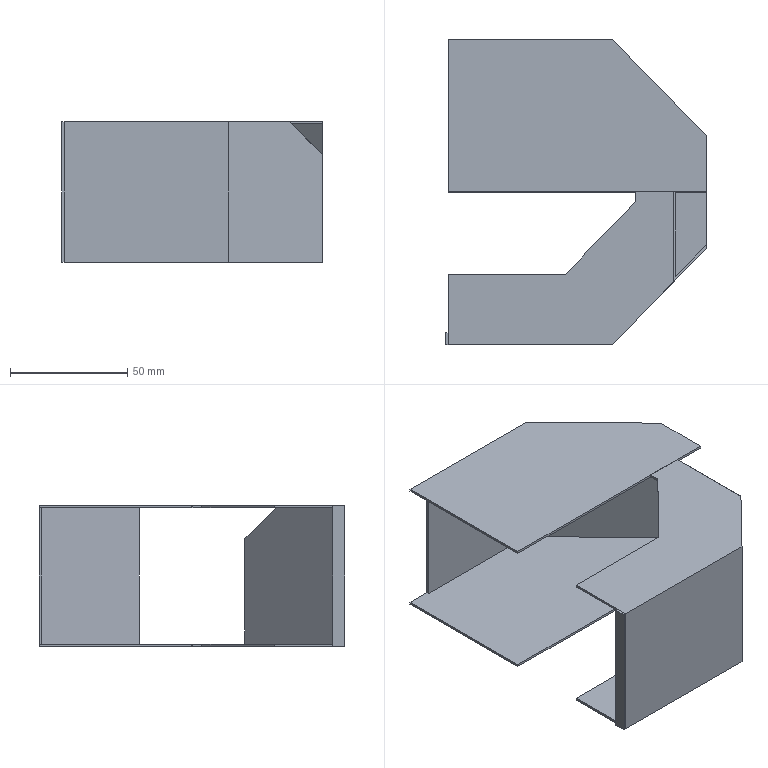Component | SolidWorks | InnerBagFunnel-1 | 3 solids | 39 faces | box 111 x 130 x 60 mm | volume 34599 mm3 | plane 39
build123d program:
from build123d import *

# Parameters (mm, degrees)
BOSS_EXTRUDE1_DEPTH      = 10
BOSS_EXTRUDE1_DEPTH_BACK = 50
SHELL1_T                 = -1
CUT_EXTRUDE1_DEPTH       = 70
SKETCH8_W                = 60
SKETCH8_H                = 5
BOSS_EXTRUDE3_DEPTH      = 1
CUT_EXTRUDE2_DEPTH       = 61
SKETCH9_W                = 10
SKETCH9_H                = 58
CUT_EXTRUDE3_DEPTH       = 10


with BuildPart() as part:
    # Sketch2 → Boss-Extrude1 (new, two sides: drawn at the far end of the back side and taken through both)
    with BuildSketch(Plane.XY.offset(-BOSS_EXTRUDE1_DEPTH_BACK)):
        Polygon((51.224, 35.92), (-18.776, 35.92), (-58.776, 76.92), (-58.776, 100.92), (51.224, 100.92), align=None)
    extrude(amount=BOSS_EXTRUDE1_DEPTH + BOSS_EXTRUDE1_DEPTH_BACK)

    # Shell1
    shell1_openings = [part.faces().sort_by_distance(p)[0] for p in [
        (-58.776, 88.92, -20),
        (-3.776, 100.92, -20),
        (51.224, 68.42, -20),
    ]]
    offset(amount=SHELL1_T, openings=shell1_openings, kind=Kind.INTERSECTION)


with BuildPart() as body_2:
    # Mirror3: mirrored copy
    add(part.part.mirror(Plane(origin=(-58.776, 100.92, 10), x_dir=(0, 0, 1), z_dir=(0, -1, 0))))

    # Sketch9 → Cut-Extrude3 (cut)
    with BuildSketch(Plane(origin=(0, 165.92, 0), x_dir=(1, 0, 0), z_dir=(0, 1, 0))):
        with Locations((46.224, 20)):
            Rectangle(SKETCH9_W, SKETCH9_H)
    extrude(amount=-CUT_EXTRUDE3_DEPTH, mode=Mode.SUBTRACT)


with BuildPart() as part_1:
    add(part.part)

    # Sketch4 → Cut-Extrude1 (cut)
    with BuildSketch(Plane.XY.offset(10)):
        Polygon((51.224, 100.92), (-28.776, 100.92), (-28.776, 96.67), (1.224, 65.92), (51.224, 65.92), align=None)
    extrude(amount=-CUT_EXTRUDE1_DEPTH, mode=Mode.SUBTRACT)

    # Sketch7 → Cut-Extrude2 (cut)
    with BuildSketch(Plane(origin=(0, 100.92, 0), x_dir=(1, 0, 0), z_dir=(0, 1, 0))):
        Polygon((-44.776, 50), (-58.776, 36), (-58.776, 50), align=None)
    extrude(amount=-CUT_EXTRUDE2_DEPTH, mode=Mode.SUBTRACT)


with BuildPart() as body_3:
    # Sketch8 → Boss-Extrude3 (new body)
    with BuildSketch(Plane(origin=(51.224, 0, 0), x_dir=(0, 0, -1), z_dir=(1, 0, 0))):
        with Locations((20, 38.42)):
            Rectangle(SKETCH8_W, SKETCH8_H)
    extrude(amount=BOSS_EXTRUDE3_DEPTH)


solid = Compound([body_2.part, part_1.part, body_3.part])

# Placed as in the assembly
solid = solid.moved(Location((-624.146, -40.37, 354.126), (-180, 0, 180)))